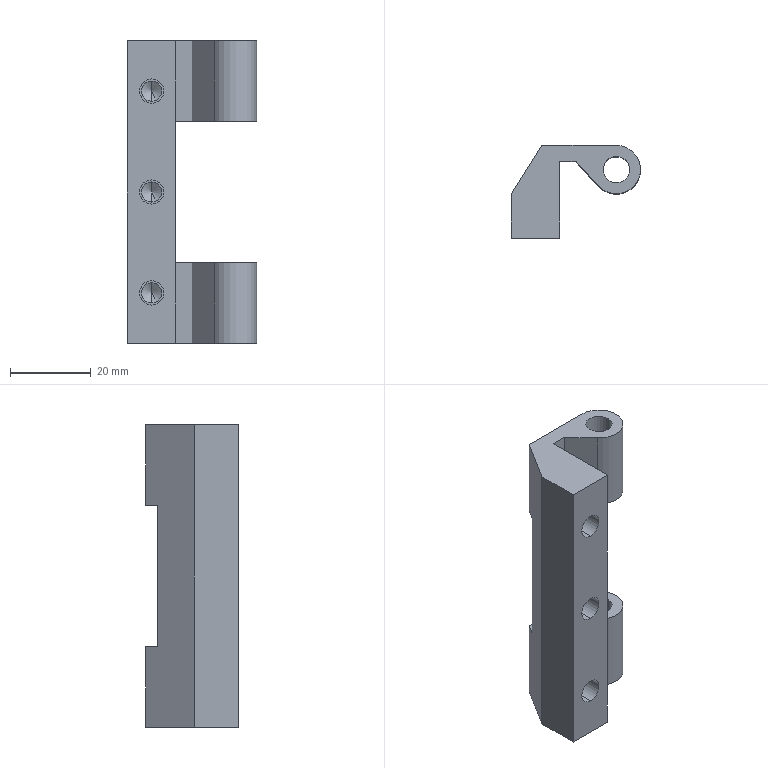Component | SolidWorks | HHL011-1RittalHinge-2 | 1 solid | 44 faces | volume 20869 mm3 | plane 20 | cylinder 18 | cone 6 | commonest cylinder face diameters 5 x6 6.01 x6 6.5 x4 12 x2